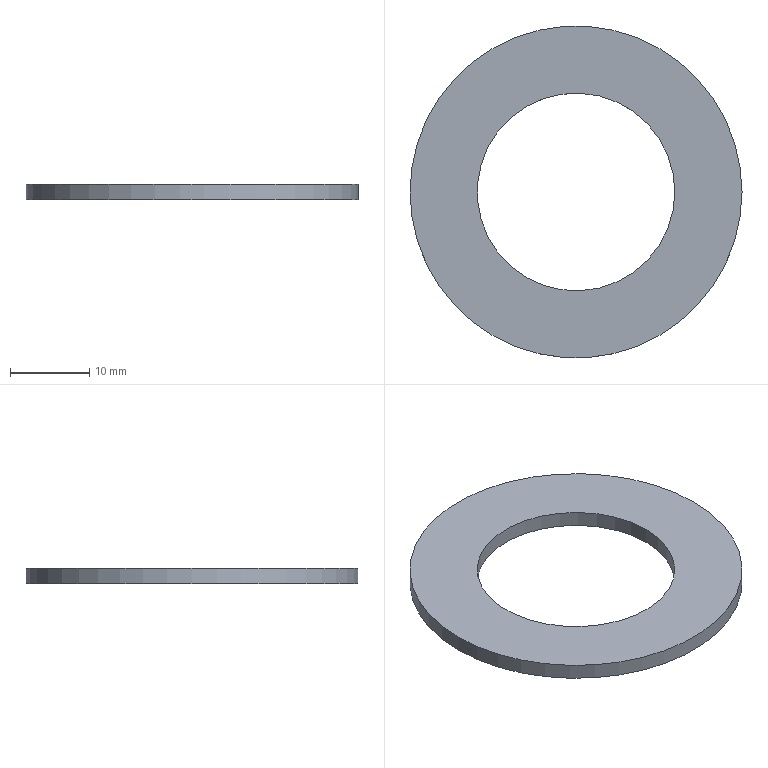Component | NX | CH3404_1-2 | 1 solid | 4 faces | box 42 x 42 x 2 mm | volume 1789 mm3 | cylinder 2 | plane 2 | commonest cylinder face diameters 42 x1 25 x1
STEP:
#1=CARTESIAN_POINT('',(0.,0.,0.));
#2=DIRECTION('',(0.,0.,1.));
#3=DIRECTION('',(1.,0.,0.));
#4=AXIS2_PLACEMENT_3D('',#1,#2,#3);
#5=CARTESIAN_POINT('',(21.,0.,12.));
#6=VERTEX_POINT('',#5);
#7=CARTESIAN_POINT('',(0.,0.,12.));
#8=DIRECTION('',(0.,0.,1.));
#9=DIRECTION('',(1.,0.,0.));
#10=AXIS2_PLACEMENT_3D('',#7,#8,#9);
#11=CIRCLE('',#10,21.);
#12=CARTESIAN_POINT('',(0.,0.,12.));
#13=DIRECTION('',(0.,0.,-1.));
#14=DIRECTION('',(-1.,0.,0.));
#15=AXIS2_PLACEMENT_3D('',#12,#13,#14);
#16=CYLINDRICAL_SURFACE('',#15,21.);
#17=CARTESIAN_POINT('',(9.425,0.));
#18=DIRECTION('',(-1.,0.));
#19=VECTOR('',#18,1.);
#20=LINE('',#17,#19);
#21=(GEOMETRIC_REPRESENTATION_CONTEXT(2)PARAMETRIC_REPRESENTATION_CONTEXT()REPRESENTATION_CONTEXT('',''));
#22=DEFINITIONAL_REPRESENTATION('',(#20),#21);
#23=PCURVE('',#16,#22);
#24=CARTESIAN_POINT('',(0.,0.,12.));
#25=DIRECTION('',(0.,0.,1.));
#26=DIRECTION('',(1.,0.,0.));
#27=AXIS2_PLACEMENT_3D('',#24,#25,#26);
#28=PLANE('',#27);
#29=CARTESIAN_POINT('',(0.,0.));
#30=DIRECTION('',(1.,0.));
#31=AXIS2_PLACEMENT_2D('',#29,#30);
#32=CIRCLE('',#31,21.);
#33=(GEOMETRIC_REPRESENTATION_CONTEXT(2)PARAMETRIC_REPRESENTATION_CONTEXT()REPRESENTATION_CONTEXT('',''));
#34=DEFINITIONAL_REPRESENTATION('',(#32),#33);
#35=PCURVE('',#28,#34);
#36=SURFACE_CURVE('',#11,(#23,#35),.PCURVE_S1.);
#37=EDGE_CURVE('',#6,#6,#36,.T.);
#38=ORIENTED_EDGE('',*,*,#37,.F.);
#39=CARTESIAN_POINT('',(21.,0.,10.));
#40=VERTEX_POINT('',#39);
#41=CARTESIAN_POINT('',(21.,0.,12.));
#42=CARTESIAN_POINT('',(21.,0.,10.));
#43=B_SPLINE_CURVE_WITH_KNOTS('',1,(#41,#42),.UNSPECIFIED.,.F.,.F.,(2,2),(0.,2.),.PIECEWISE_BEZIER_KNOTS.);
#44=CARTESIAN_POINT('',(9.425,0.));
#45=DIRECTION('',(0.,1.));
#46=VECTOR('',#45,1.);
#47=LINE('',#44,#46);
#48=(GEOMETRIC_REPRESENTATION_CONTEXT(2)PARAMETRIC_REPRESENTATION_CONTEXT()REPRESENTATION_CONTEXT('',''));
#49=DEFINITIONAL_REPRESENTATION('',(#47),#48);
#50=PCURVE('',#16,#49);
#51=CARTESIAN_POINT('',(3.142,0.));
#52=DIRECTION('',(0.,1.));
#53=VECTOR('',#52,1.);
#54=LINE('',#51,#53);
#55=(GEOMETRIC_REPRESENTATION_CONTEXT(2)PARAMETRIC_REPRESENTATION_CONTEXT()REPRESENTATION_CONTEXT('',''));
#56=DEFINITIONAL_REPRESENTATION('',(#54),#55);
#57=PCURVE('',#16,#56);
#58=SEAM_CURVE('',#43,(#50,#57),.PCURVE_S1.);
#59=EDGE_CURVE('',#6,#40,#58,.T.);
#60=ORIENTED_EDGE('',*,*,#59,.T.);
#61=CARTESIAN_POINT('',(0.,0.,10.));
#62=DIRECTION('',(0.,0.,1.));
#63=DIRECTION('',(1.,0.,0.));
#64=AXIS2_PLACEMENT_3D('',#61,#62,#63);
#65=CIRCLE('',#64,21.);
#66=CARTESIAN_POINT('',(9.425,2.));
#67=DIRECTION('',(-1.,0.));
#68=VECTOR('',#67,1.);
#69=LINE('',#66,#68);
#70=(GEOMETRIC_REPRESENTATION_CONTEXT(2)PARAMETRIC_REPRESENTATION_CONTEXT()REPRESENTATION_CONTEXT('',''));
#71=DEFINITIONAL_REPRESENTATION('',(#69),#70);
#72=PCURVE('',#16,#71);
#73=CARTESIAN_POINT('',(0.,0.,10.));
#74=DIRECTION('',(0.,0.,1.));
#75=DIRECTION('',(1.,0.,0.));
#76=AXIS2_PLACEMENT_3D('',#73,#74,#75);
#77=PLANE('',#76);
#78=CARTESIAN_POINT('',(0.,0.));
#79=DIRECTION('',(1.,0.));
#80=AXIS2_PLACEMENT_2D('',#78,#79);
#81=CIRCLE('',#80,21.);
#82=(GEOMETRIC_REPRESENTATION_CONTEXT(2)PARAMETRIC_REPRESENTATION_CONTEXT()REPRESENTATION_CONTEXT('',''));
#83=DEFINITIONAL_REPRESENTATION('',(#81),#82);
#84=PCURVE('',#77,#83);
#85=SURFACE_CURVE('',#65,(#72,#84),.PCURVE_S1.);
#86=EDGE_CURVE('',#40,#40,#85,.T.);
#87=ORIENTED_EDGE('',*,*,#86,.T.);
#88=ORIENTED_EDGE('',*,*,#59,.F.);
#89=EDGE_LOOP('',(#38,#60,#87,#88));
#90=FACE_BOUND('',#89,.T.);
#91=ADVANCED_FACE('',(#90),#16,.T.);
#92=CARTESIAN_POINT('',(12.5,0.,12.));
#93=VERTEX_POINT('',#92);
#94=CARTESIAN_POINT('',(0.,0.,12.));
#95=DIRECTION('',(0.,0.,1.));
#96=DIRECTION('',(1.,0.,0.));
#97=AXIS2_PLACEMENT_3D('',#94,#95,#96);
#98=CIRCLE('',#97,12.5);
#99=CARTESIAN_POINT('',(0.,0.,12.));
#100=DIRECTION('',(0.,0.,-1.));
#101=DIRECTION('',(-1.,0.,0.));
#102=AXIS2_PLACEMENT_3D('',#99,#100,#101);
#103=CYLINDRICAL_SURFACE('',#102,12.5);
#104=CARTESIAN_POINT('',(9.425,0.));
#105=DIRECTION('',(-1.,0.));
#106=VECTOR('',#105,1.);
#107=LINE('',#104,#106);
#108=(GEOMETRIC_REPRESENTATION_CONTEXT(2)PARAMETRIC_REPRESENTATION_CONTEXT()REPRESENTATION_CONTEXT('',''));
#109=DEFINITIONAL_REPRESENTATION('',(#107),#108);
#110=PCURVE('',#103,#109);
#111=CARTESIAN_POINT('',(0.,0.));
#112=DIRECTION('',(1.,0.));
#113=AXIS2_PLACEMENT_2D('',#111,#112);
#114=CIRCLE('',#113,12.5);
#115=(GEOMETRIC_REPRESENTATION_CONTEXT(2)PARAMETRIC_REPRESENTATION_CONTEXT()REPRESENTATION_CONTEXT('',''));
#116=DEFINITIONAL_REPRESENTATION('',(#114),#115);
#117=PCURVE('',#28,#116);
#118=SURFACE_CURVE('',#98,(#110,#117),.PCURVE_S1.);
#119=EDGE_CURVE('',#93,#93,#118,.T.);
#120=ORIENTED_EDGE('',*,*,#119,.F.);
#121=CARTESIAN_POINT('',(12.5,0.,10.));
#122=VERTEX_POINT('',#121);
#123=CARTESIAN_POINT('',(12.5,0.,12.));
#124=CARTESIAN_POINT('',(12.5,0.,10.));
#125=B_SPLINE_CURVE_WITH_KNOTS('',1,(#123,#124),.UNSPECIFIED.,.F.,.F.,(2,2),(0.,2.),.PIECEWISE_BEZIER_KNOTS.);
#126=CARTESIAN_POINT('',(9.425,0.));
#127=DIRECTION('',(0.,1.));
#128=VECTOR('',#127,1.);
#129=LINE('',#126,#128);
#130=(GEOMETRIC_REPRESENTATION_CONTEXT(2)PARAMETRIC_REPRESENTATION_CONTEXT()REPRESENTATION_CONTEXT('',''));
#131=DEFINITIONAL_REPRESENTATION('',(#129),#130);
#132=PCURVE('',#103,#131);
#133=CARTESIAN_POINT('',(3.142,0.));
#134=DIRECTION('',(0.,1.));
#135=VECTOR('',#134,1.);
#136=LINE('',#133,#135);
#137=(GEOMETRIC_REPRESENTATION_CONTEXT(2)PARAMETRIC_REPRESENTATION_CONTEXT()REPRESENTATION_CONTEXT('',''));
#138=DEFINITIONAL_REPRESENTATION('',(#136),#137);
#139=PCURVE('',#103,#138);
#140=SEAM_CURVE('',#125,(#132,#139),.PCURVE_S1.);
#141=EDGE_CURVE('',#93,#122,#140,.T.);
#142=ORIENTED_EDGE('',*,*,#141,.T.);
#143=CARTESIAN_POINT('',(0.,0.,10.));
#144=DIRECTION('',(0.,0.,1.));
#145=DIRECTION('',(1.,0.,0.));
#146=AXIS2_PLACEMENT_3D('',#143,#144,#145);
#147=CIRCLE('',#146,12.5);
#148=CARTESIAN_POINT('',(9.425,2.));
#149=DIRECTION('',(-1.,0.));
#150=VECTOR('',#149,1.);
#151=LINE('',#148,#150);
#152=(GEOMETRIC_REPRESENTATION_CONTEXT(2)PARAMETRIC_REPRESENTATION_CONTEXT()REPRESENTATION_CONTEXT('',''));
#153=DEFINITIONAL_REPRESENTATION('',(#151),#152);
#154=PCURVE('',#103,#153);
#155=CARTESIAN_POINT('',(0.,0.));
#156=DIRECTION('',(1.,0.));
#157=AXIS2_PLACEMENT_2D('',#155,#156);
#158=CIRCLE('',#157,12.5);
#159=(GEOMETRIC_REPRESENTATION_CONTEXT(2)PARAMETRIC_REPRESENTATION_CONTEXT()REPRESENTATION_CONTEXT('',''));
#160=DEFINITIONAL_REPRESENTATION('',(#158),#159);
#161=PCURVE('',#77,#160);
#162=SURFACE_CURVE('',#147,(#154,#161),.PCURVE_S1.);
#163=EDGE_CURVE('',#122,#122,#162,.T.);
#164=ORIENTED_EDGE('',*,*,#163,.T.);
#165=ORIENTED_EDGE('',*,*,#141,.F.);
#166=EDGE_LOOP('',(#120,#142,#164,#165));
#167=FACE_BOUND('',#166,.F.);
#168=ADVANCED_FACE('',(#167),#103,.F.);
#169=ORIENTED_EDGE('',*,*,#37,.T.);
#170=EDGE_LOOP('',(#169));
#171=FACE_BOUND('',#170,.T.);
#172=ORIENTED_EDGE('',*,*,#119,.F.);
#173=EDGE_LOOP('',(#172));
#174=FACE_BOUND('',#173,.T.);
#175=ADVANCED_FACE('',(#171,#174),#28,.T.);
#176=ORIENTED_EDGE('',*,*,#86,.F.);
#177=EDGE_LOOP('',(#176));
#178=FACE_BOUND('',#177,.T.);
#179=ORIENTED_EDGE('',*,*,#163,.T.);
#180=EDGE_LOOP('',(#179));
#181=FACE_BOUND('',#180,.T.);
#182=ADVANCED_FACE('',(#178,#181),#77,.F.);
#183=CLOSED_SHELL('',(#91,#168,#175,#182));
#184=MANIFOLD_SOLID_BREP('',#183);
#185=(LENGTH_UNIT()NAMED_UNIT(*)SI_UNIT(.MILLI.,.METRE.));
#186=UNCERTAINTY_MEASURE_WITH_UNIT(LENGTH_MEASURE(0.00001),#185,'','');
#187=(NAMED_UNIT(*)PLANE_ANGLE_UNIT()SI_UNIT($,.RADIAN.));
#188=(NAMED_UNIT(*)SI_UNIT($,.STERADIAN.)SOLID_ANGLE_UNIT());
#189=(GEOMETRIC_REPRESENTATION_CONTEXT(3)GLOBAL_UNCERTAINTY_ASSIGNED_CONTEXT((#186))GLOBAL_UNIT_ASSIGNED_CONTEXT((#185,#187,#188))REPRESENTATION_CONTEXT('',''));
#190=ADVANCED_BREP_SHAPE_REPRESENTATION('',(#4,#184),#189);